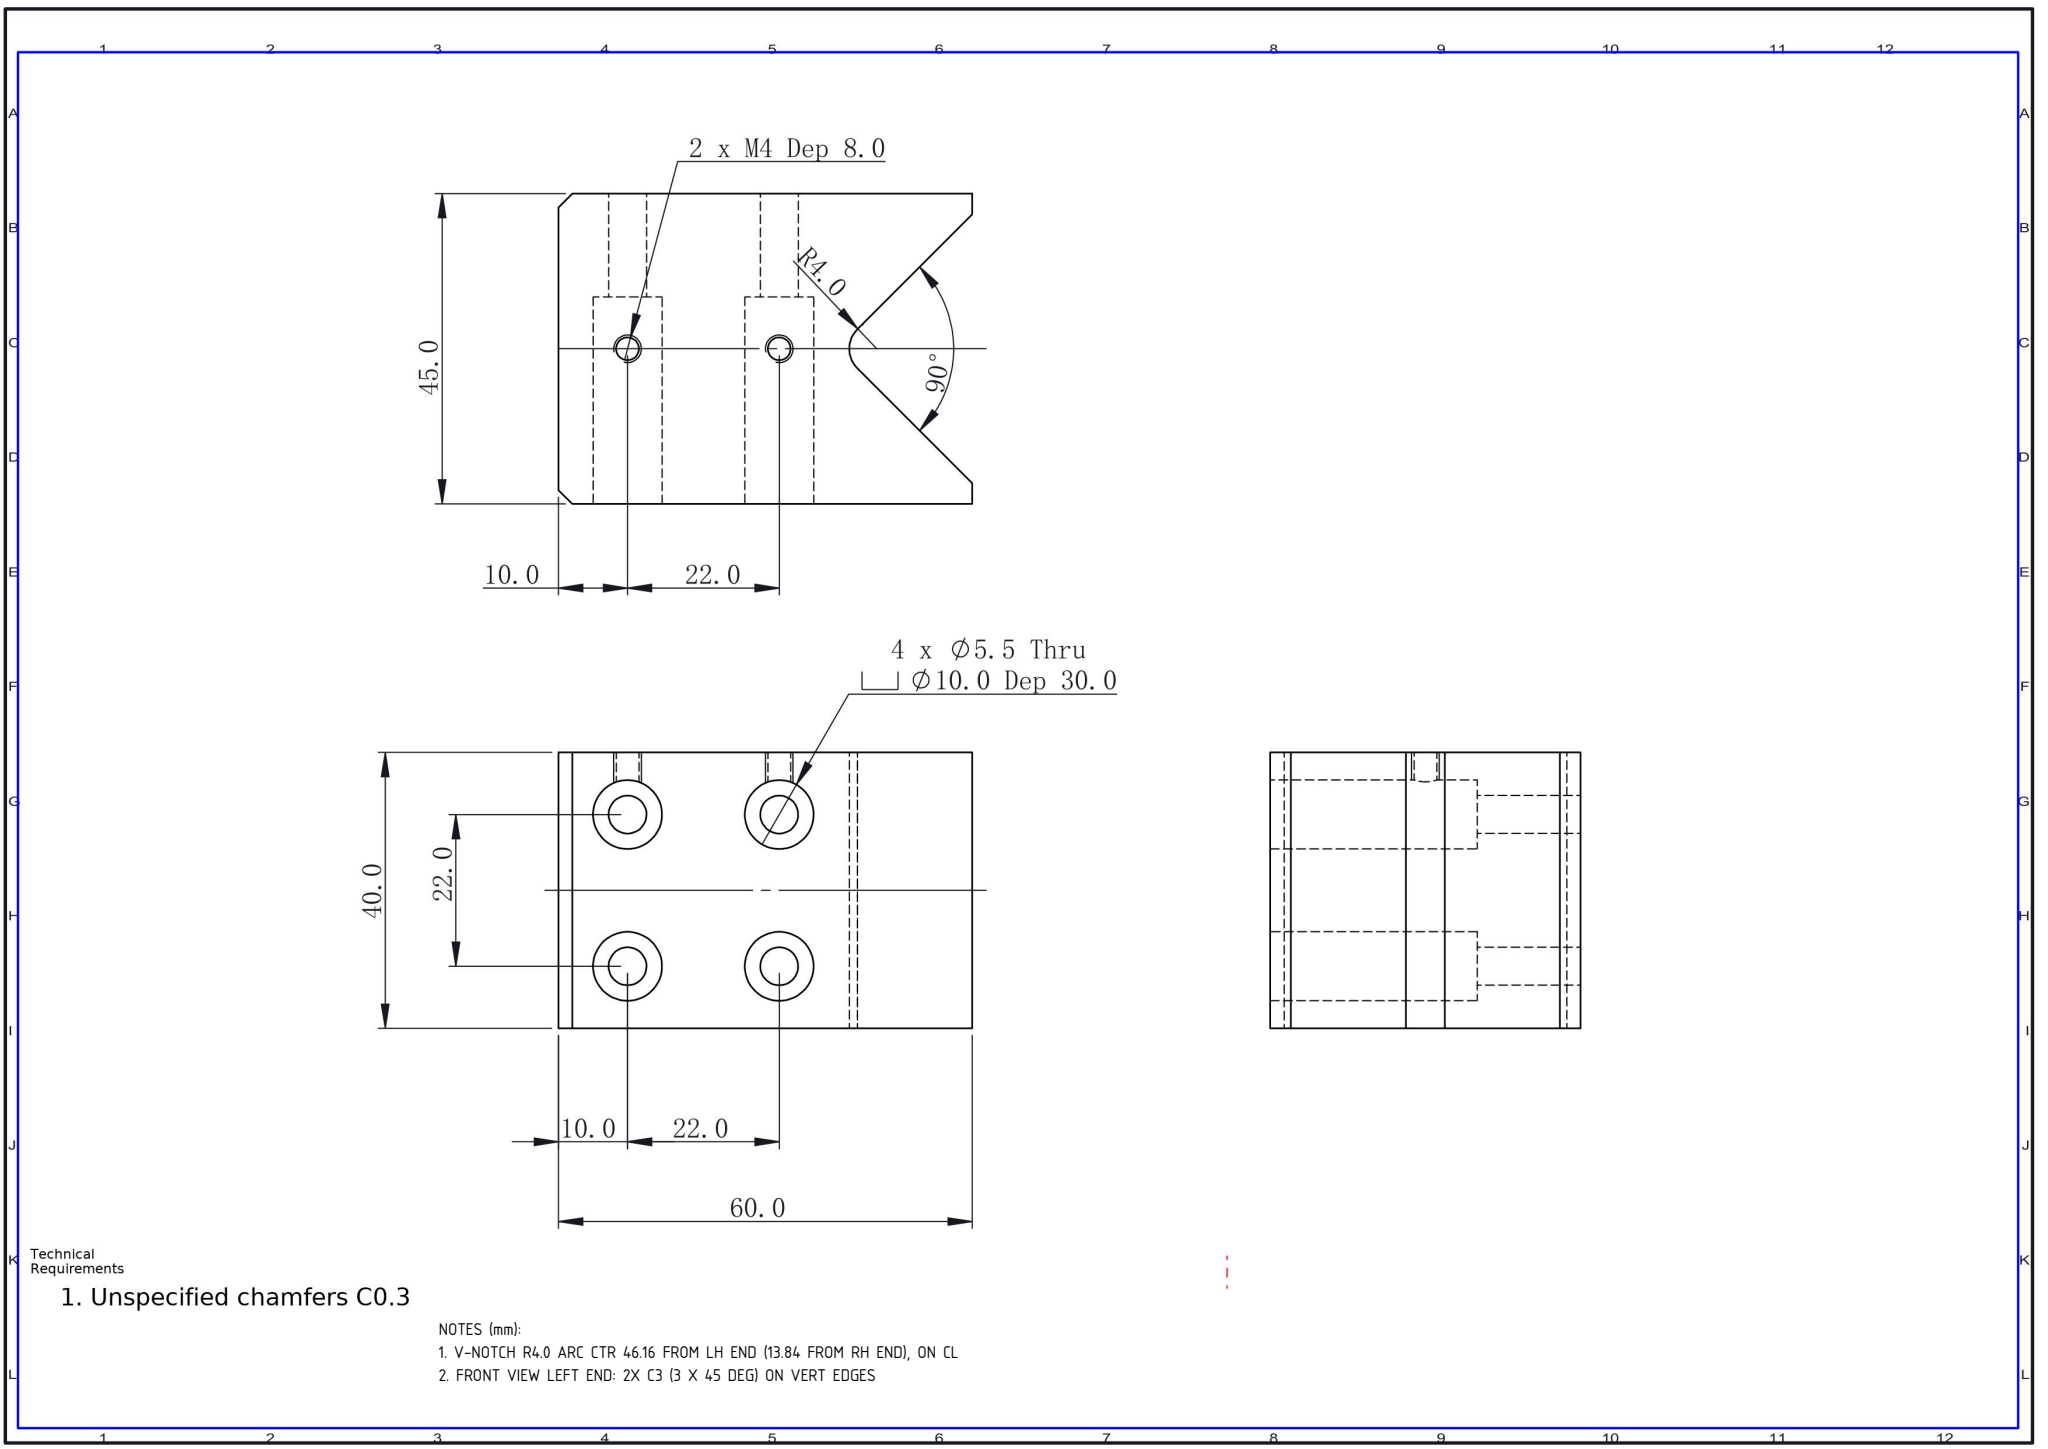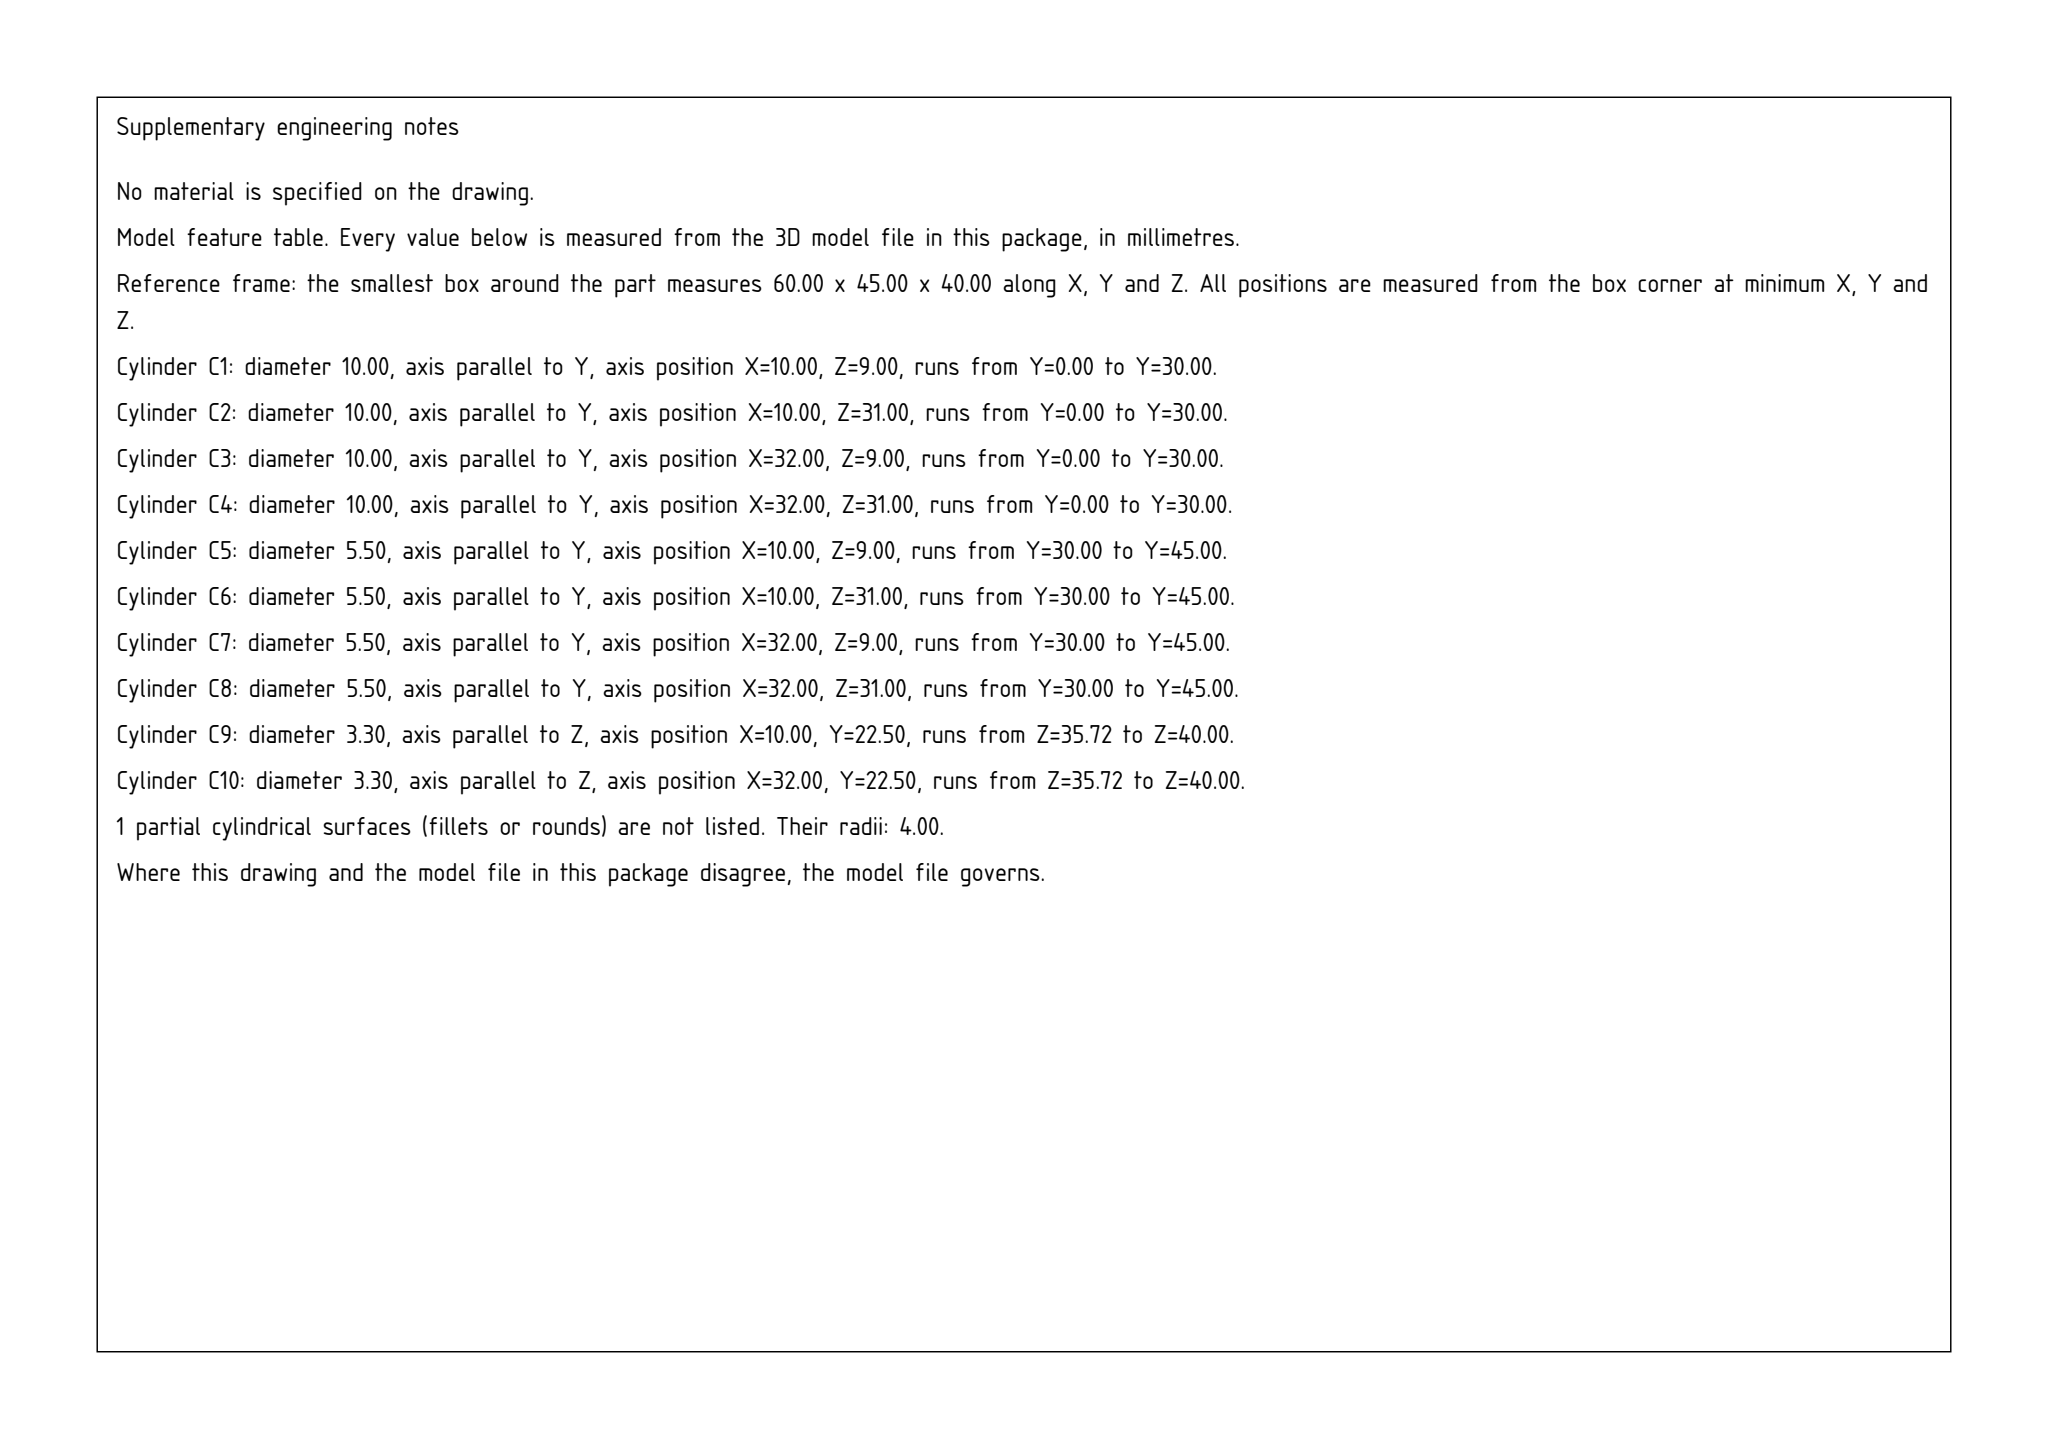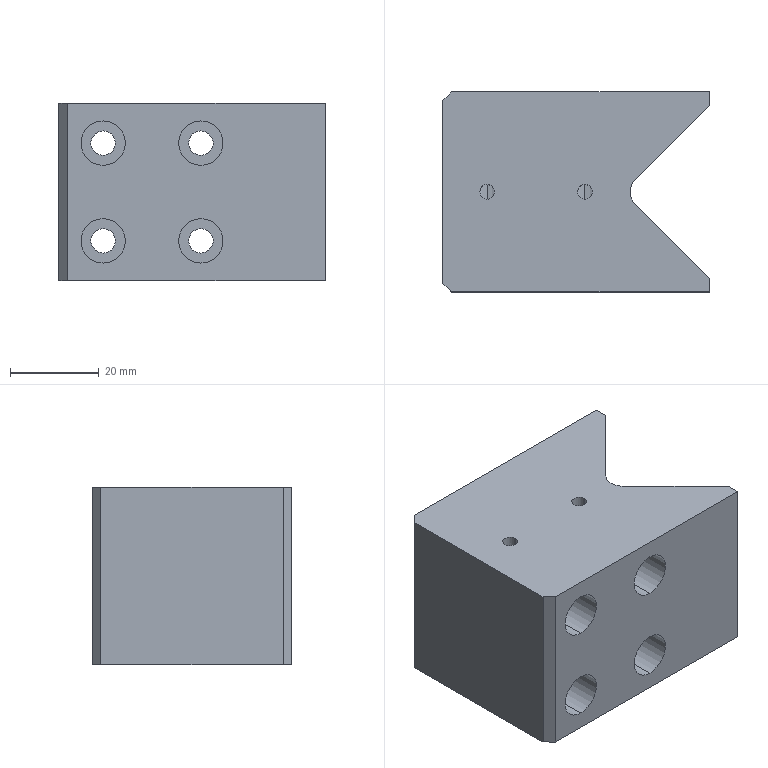Part | SolidWorks | mm | 1 solid | 36 faces | box 60 x 45 x 40 mm | volume 81847 mm3 | cylinder 21 | plane 15 | commonest cylinder face diameters 10 x8 5.5 x8 3.3 x4 8 x1
Drawing notes:
V-NOTCH R4.0 ARC CTR 46.16 FROM LH END (13.84 FROM RH END), ON CL | from the solid: cylinder dia 8.0 (R4.0) axis z at [46.16, 22.5], length 40.0 = full thickness; bbox X 60.0
FRONT VIEW LEFT END: 2X C3 (3 X 45 DEG) ON VERT EDGES | from the solid: Left end face x=0 meets y=0 and y=45 faces via 45 deg cut planes (not axis-aligned, so absent from axis_planes); measured cut 3 mm, overrides note C0.3
build123d program:
from build123d import *

# Parameters (mm, degrees)
BOSS_EXTRUDE1_DEPTH                             = 40
M5_HEX_SOCKET_HEAD_CAP_SCREW_CBORE1_D           = 5.5
M5_HEX_SOCKET_HEAD_CAP_SCREW_CBORE1_CBORE_D     = 10
M5_HEX_SOCKET_HEAD_CAP_SCREW_CBORE1_CBORE_DEPTH = 30
M4_TAPPED_HOLE1_D                               = 3.3
M4_TAPPED_HOLE1_DEPTH                           = 10.1
M4_TAPPED_HOLE1_TIP                             = 0.9914
CHAMFER1_SIZE                                   = 2
FILLET1_R                                       = 4


with BuildPart() as part:
    # Sketch1 → Boss-Extrude1 (new body)
    with BuildSketch(Plane.XY):
        Polygon((60, 42), (40.5, 22.5), (60, 3), (60, 0), (0, 0), (0, 45), (60, 45), align=None)
    extrude(amount=BOSS_EXTRUDE1_DEPTH)

    # M5 Hex Socket Head Cap Screw CBORE1 (through all)
    with Locations(Plane(origin=(0, 0, 0), x_dir=(-1, 0, 0), z_dir=(0, -1, 0))):
        with Locations((-10, -31), (-32, -31), (-10, -9), (-32, -9)):
            CounterBoreHole(M5_HEX_SOCKET_HEAD_CAP_SCREW_CBORE1_D / 2, M5_HEX_SOCKET_HEAD_CAP_SCREW_CBORE1_CBORE_D / 2, M5_HEX_SOCKET_HEAD_CAP_SCREW_CBORE1_CBORE_DEPTH)

    # M4 Tapped Hole1
    with Locations(Plane.XY.offset(40)):
        with Locations((10, 22.5), (32, 22.5)):
            Hole(M4_TAPPED_HOLE1_D / 2, depth=M4_TAPPED_HOLE1_DEPTH)
            with Locations((0, 0, -(M4_TAPPED_HOLE1_DEPTH + M4_TAPPED_HOLE1_TIP / 2))):  # 118° drill point
                Cone(0, M4_TAPPED_HOLE1_D / 2, M4_TAPPED_HOLE1_TIP, mode=Mode.SUBTRACT)

    # Chamfer1
    chamfer1_edges = [part.edges().sort_by_distance(p)[0] for p in [
        (0, 45, 20),
        (0, 0, 20),
    ]]
    chamfer(chamfer1_edges, length=CHAMFER1_SIZE)

    # Fillet1
    fillet1_edges = [part.edges().sort_by_distance(p)[0] for p in [
        (40.5, 22.5, 20),
    ]]
    fillet(fillet1_edges, radius=FILLET1_R)


solid = part.part